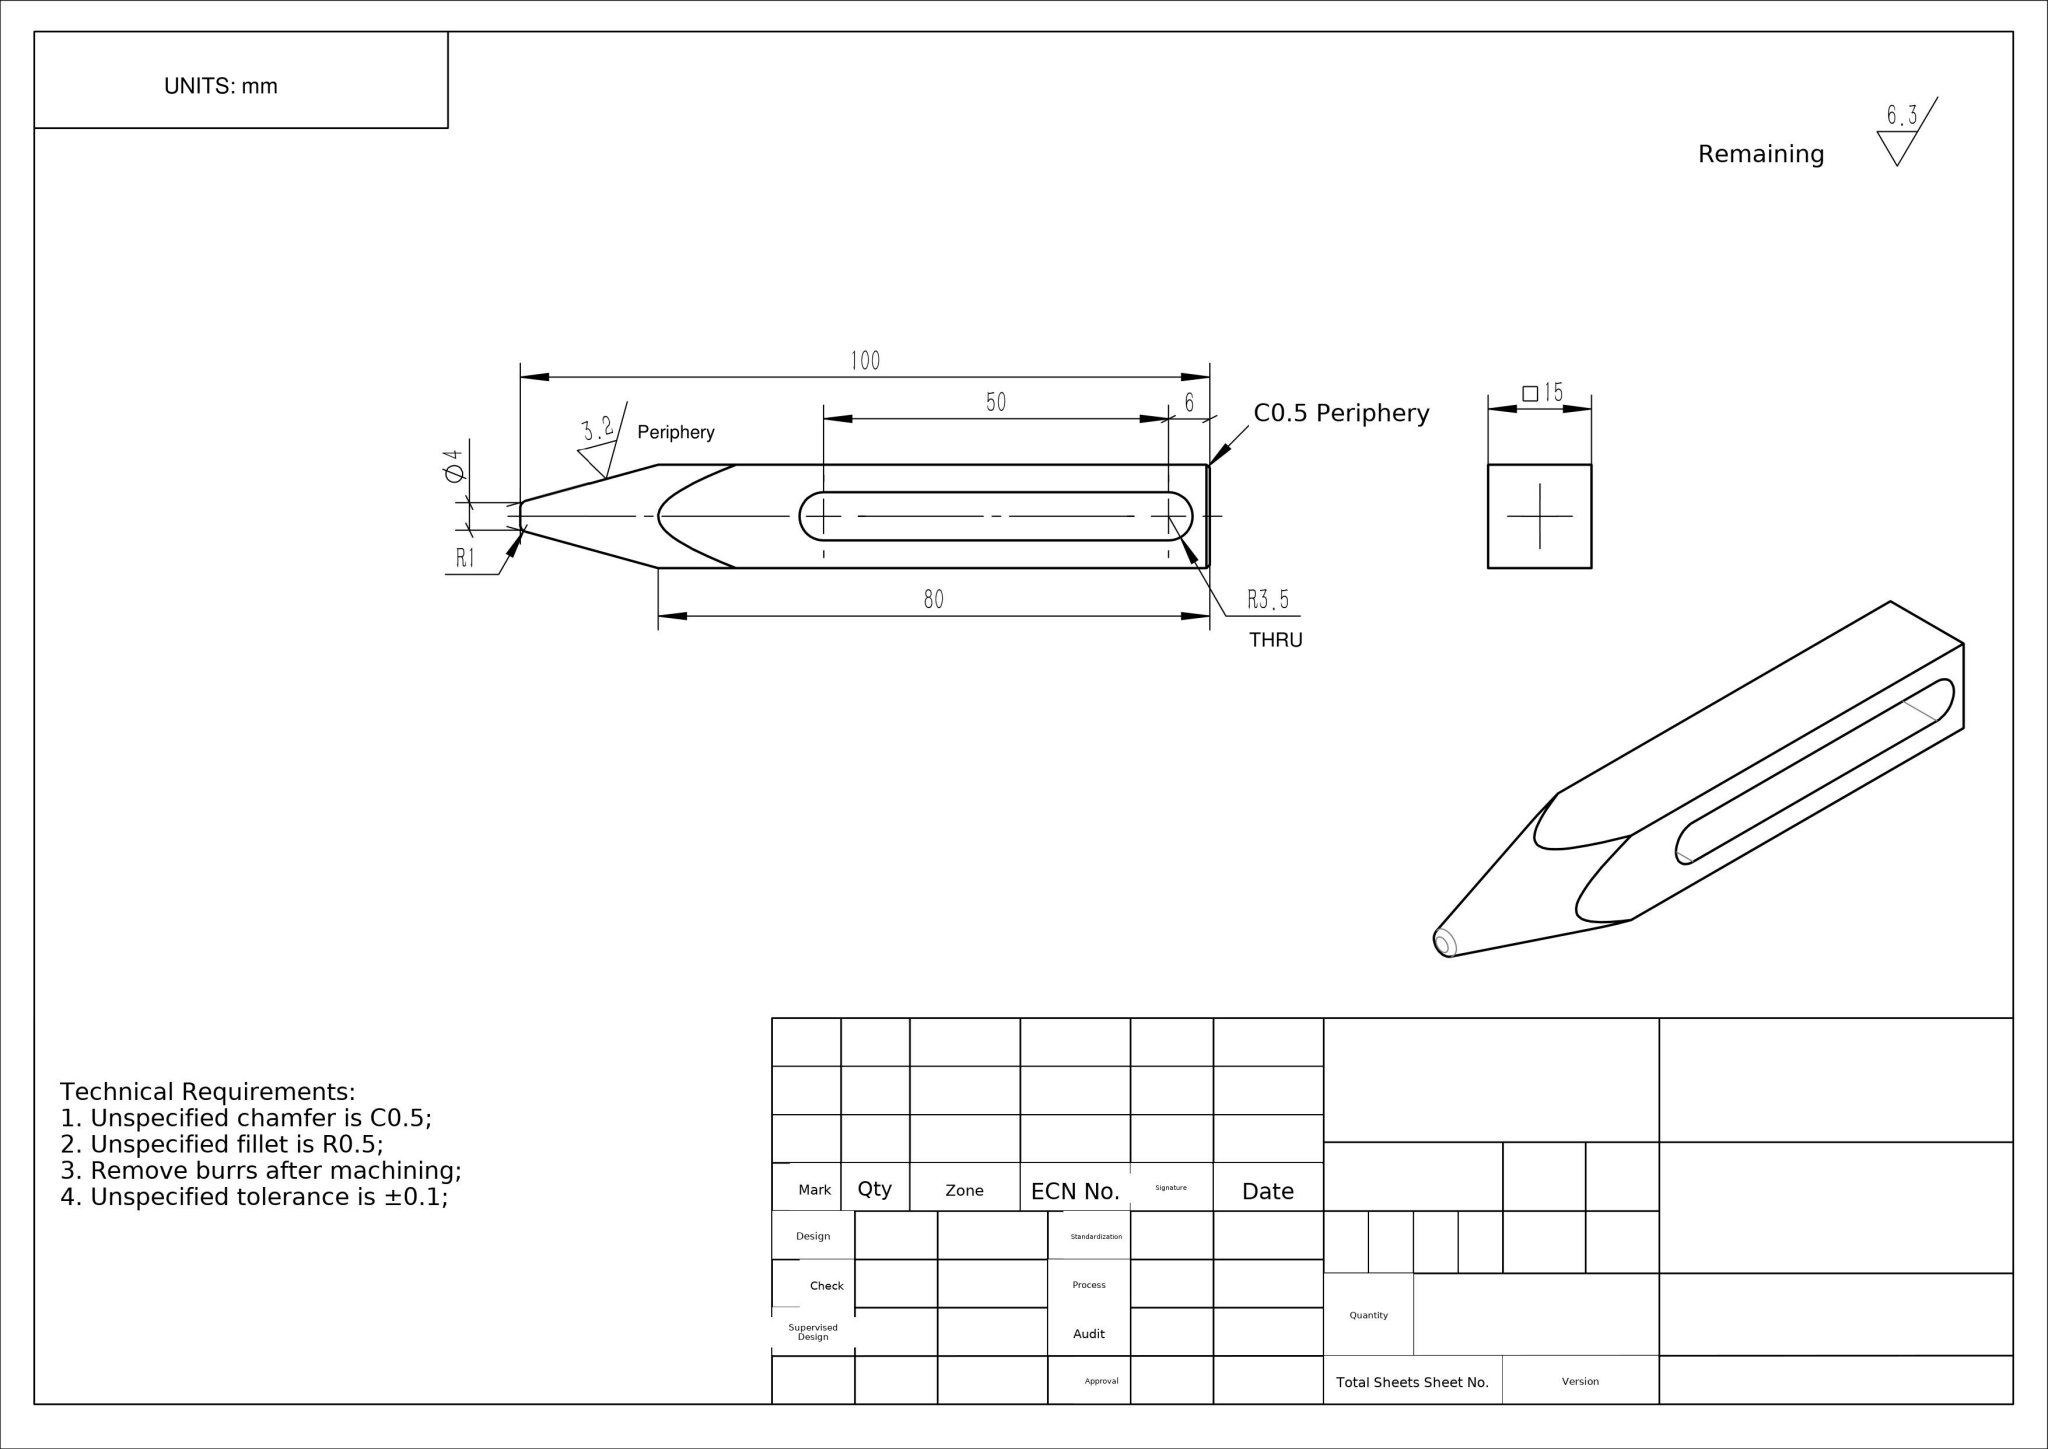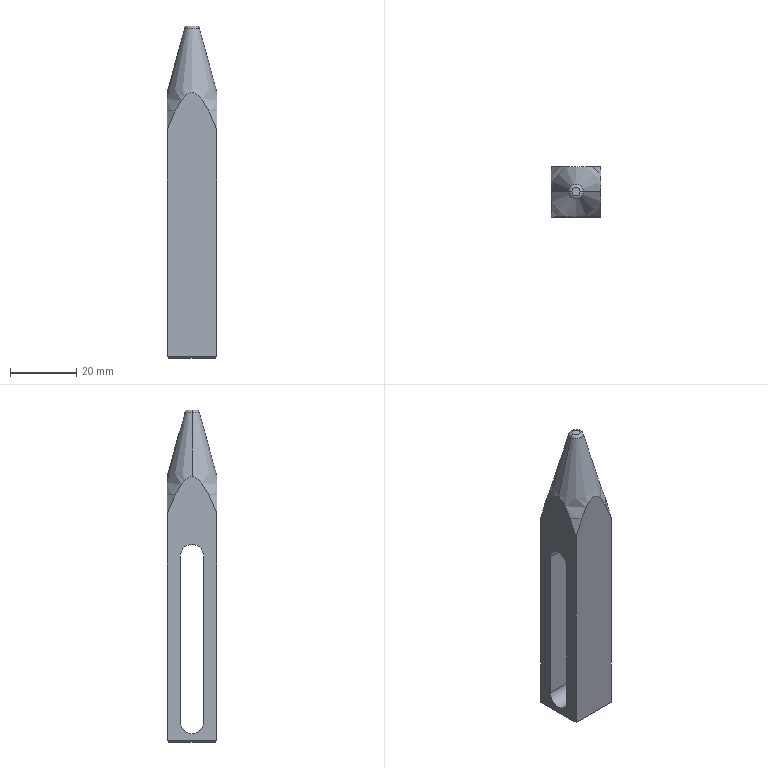Part | NX | mm | 1 solid | 19 faces | box 15 x 15 x 100 mm | volume 13574 mm3 | plane 12 | cylinder 3 | torus 2 | cone 2 | commonest cylinder face diameters 7 x3
STEP:
#1=COLOUR_RGB('',0.698,0.698,0.698);
#2=FILL_AREA_STYLE_COLOUR('',#1);
#3=FILL_AREA_STYLE('',(#2));
#4=SURFACE_STYLE_FILL_AREA(#3);
#5=SURFACE_SIDE_STYLE('',(#4));
#6=SURFACE_STYLE_USAGE(.BOTH.,#5);
#7=PRESENTATION_STYLE_ASSIGNMENT((#6));
#8=CARTESIAN_POINT('',(7.5,0.,9.5));
#9=VERTEX_POINT('',#8);
#10=CARTESIAN_POINT('',(7.5,3.5,6.));
#11=VERTEX_POINT('',#10);
#12=CARTESIAN_POINT('',(7.5,0.,6.));
#13=DIRECTION('',(-1.,0.,0.));
#14=DIRECTION('',(0.,0.,1.));
#15=AXIS2_PLACEMENT_3D('',#12,#13,#14);
#16=CIRCLE('',#15,3.5);
#17=EDGE_CURVE('',#9,#11,#16,.T.);
#18=ORIENTED_EDGE('',*,*,#17,.F.);
#19=CARTESIAN_POINT('',(-7.5,0.,9.5));
#20=VERTEX_POINT('',#19);
#21=CARTESIAN_POINT('',(7.5,0.,9.5));
#22=DIRECTION('',(-1.,0.,0.));
#23=VECTOR('',#22,1000.);
#24=LINE('',#21,#23);
#25=EDGE_CURVE('',#9,#20,#24,.T.);
#26=ORIENTED_EDGE('',*,*,#25,.T.);
#27=CARTESIAN_POINT('',(-7.5,3.5,6.));
#28=VERTEX_POINT('',#27);
#29=CARTESIAN_POINT('',(-7.5,0.,6.));
#30=DIRECTION('',(-1.,0.,0.));
#31=DIRECTION('',(0.,0.,1.));
#32=AXIS2_PLACEMENT_3D('',#29,#30,#31);
#33=CIRCLE('',#32,3.5);
#34=EDGE_CURVE('',#20,#28,#33,.T.);
#35=ORIENTED_EDGE('',*,*,#34,.T.);
#36=CARTESIAN_POINT('',(7.5,3.5,6.));
#37=DIRECTION('',(-1.,0.,0.));
#38=VECTOR('',#37,1000.);
#39=LINE('',#36,#38);
#40=EDGE_CURVE('',#11,#28,#39,.T.);
#41=ORIENTED_EDGE('',*,*,#40,.F.);
#42=EDGE_LOOP('',(#18,#26,#35,#41));
#43=FACE_OUTER_BOUND('',#42,.T.);
#44=CARTESIAN_POINT('',(7.5,0.,6.));
#45=DIRECTION('',(-1.,0.,0.));
#46=DIRECTION('',(0.,0.,1.));
#47=AXIS2_PLACEMENT_3D('',#44,#45,#46);
#48=CYLINDRICAL_SURFACE('',#47,3.5);
#49=ADVANCED_FACE('',(#43),#48,.F.);
#50=CARTESIAN_POINT('',(-2.202,0.,49.265));
#51=VERTEX_POINT('',#50);
#52=CARTESIAN_POINT('',(2.202,0.,49.265));
#53=VERTEX_POINT('',#52);
#54=CARTESIAN_POINT('',(0.,0.,49.265));
#55=DIRECTION('',(0.,0.,-1.));
#56=DIRECTION('',(-1.,0.,0.));
#57=AXIS2_PLACEMENT_3D('',#54,#55,#56);
#58=CIRCLE('',#57,2.202);
#59=EDGE_CURVE('',#51,#53,#58,.T.);
#60=ORIENTED_EDGE('',*,*,#59,.F.);
#61=CARTESIAN_POINT('',(-1.238,0.,50.));
#62=VERTEX_POINT('',#61);
#63=CARTESIAN_POINT('',(-1.238,0.,49.));
#64=DIRECTION('',(0.,1.,0.));
#65=DIRECTION('',(-1.,0.,0.));
#66=AXIS2_PLACEMENT_3D('',#63,#64,#65);
#67=CIRCLE('',#66,1.);
#68=EDGE_CURVE('',#51,#62,#67,.T.);
#69=ORIENTED_EDGE('',*,*,#68,.T.);
#70=CARTESIAN_POINT('',(1.238,0.,50.));
#71=VERTEX_POINT('',#70);
#72=CARTESIAN_POINT('',(0.,0.,50.));
#73=DIRECTION('',(0.,0.,1.));
#74=DIRECTION('',(1.,0.,0.));
#75=AXIS2_PLACEMENT_3D('',#72,#73,#74);
#76=CIRCLE('',#75,1.238);
#77=EDGE_CURVE('',#71,#62,#76,.T.);
#78=ORIENTED_EDGE('',*,*,#77,.F.);
#79=CARTESIAN_POINT('',(1.238,0.,49.));
#80=DIRECTION('',(0.,-1.,0.));
#81=DIRECTION('',(0.,0.,-1.));
#82=AXIS2_PLACEMENT_3D('',#79,#80,#81);
#83=CIRCLE('',#82,1.);
#84=EDGE_CURVE('',#53,#71,#83,.T.);
#85=ORIENTED_EDGE('',*,*,#84,.F.);
#86=EDGE_LOOP('',(#60,#69,#78,#85));
#87=FACE_OUTER_BOUND('',#86,.T.);
#88=CARTESIAN_POINT('',(0.,0.,49.));
#89=DIRECTION('',(0.,0.,1.));
#90=DIRECTION('',(1.,0.,0.));
#91=AXIS2_PLACEMENT_3D('',#88,#89,#90);
#92=TOROIDAL_SURFACE('',#91,1.238,1.);
#93=ADVANCED_FACE('',(#87),#92,.T.);
#94=ORIENTED_EDGE('',*,*,#59,.T.);
#95=CARTESIAN_POINT('',(7.5,0.,30.));
#96=VERTEX_POINT('',#95);
#97=CARTESIAN_POINT('',(12.,0.,13.636));
#98=DIRECTION('',(0.2652,0.,-0.9642));
#99=VECTOR('',#98,1000.);
#100=LINE('',#97,#99);
#101=EDGE_CURVE('',#53,#96,#100,.T.);
#102=ORIENTED_EDGE('',*,*,#101,.T.);
#103=CARTESIAN_POINT('',(7.5,7.5,18.703));
#104=VERTEX_POINT('',#103);
#105=CARTESIAN_POINT('',(7.5,7.5,18.703));
#106=CARTESIAN_POINT('',(7.5,7.077,19.79));
#107=CARTESIAN_POINT('',(7.5,6.64,20.871));
#108=CARTESIAN_POINT('',(7.5,5.714,23.011));
#109=CARTESIAN_POINT('',(7.5,5.228,24.07));
#110=CARTESIAN_POINT('',(7.5,4.421,25.626));
#111=CARTESIAN_POINT('',(7.5,4.139,26.139));
#112=CARTESIAN_POINT('',(7.5,3.53,27.146));
#113=CARTESIAN_POINT('',(7.5,3.207,27.637));
#114=CARTESIAN_POINT('',(7.5,2.669,28.33));
#115=CARTESIAN_POINT('',(7.5,2.482,28.555));
#116=CARTESIAN_POINT('',(7.5,2.078,28.981));
#117=CARTESIAN_POINT('',(7.5,1.861,29.186));
#118=CARTESIAN_POINT('',(7.5,1.392,29.546));
#119=CARTESIAN_POINT('',(7.5,1.142,29.704));
#120=CARTESIAN_POINT('',(7.5,0.7287,29.876));
#121=CARTESIAN_POINT('',(7.5,0.5877,29.921));
#122=CARTESIAN_POINT('',(7.5,0.2981,29.984));
#123=CARTESIAN_POINT('',(7.5,0.1479,30.));
#124=CARTESIAN_POINT('',(7.5,0.,30.));
#125=B_SPLINE_CURVE_WITH_KNOTS('',3,(#105,#106,#107,#108,#109,#110,#111,#112,#113,#114,#115,#116,#117,#118,#119,#120,#121,#122,#123,#124),.UNSPECIFIED.,.F.,.F.,(4,2,2,2,2,2,2,2,2,4),(0.05853,0.06203,0.06553,0.06728,0.06903,0.06991,0.07078,0.07166,0.0721,0.07253),.UNSPECIFIED.);
#126=EDGE_CURVE('',#104,#96,#125,.T.);
#127=ORIENTED_EDGE('',*,*,#126,.F.);
#128=CARTESIAN_POINT('',(-7.5,7.5,18.703));
#129=VERTEX_POINT('',#128);
#130=CARTESIAN_POINT('',(-7.5,7.5,18.703));
#131=CARTESIAN_POINT('',(-7.076,7.5,19.794));
#132=CARTESIAN_POINT('',(-6.636,7.5,20.881));
#133=CARTESIAN_POINT('',(-5.705,7.5,23.032));
#134=CARTESIAN_POINT('',(-5.215,7.5,24.098));
#135=CARTESIAN_POINT('',(-4.403,7.5,25.658));
#136=CARTESIAN_POINT('',(-4.121,7.5,26.17));
#137=CARTESIAN_POINT('',(-3.516,7.5,27.168));
#138=CARTESIAN_POINT('',(-3.194,7.5,27.655));
#139=CARTESIAN_POINT('',(-2.655,7.5,28.348));
#140=CARTESIAN_POINT('',(-2.466,7.5,28.573));
#141=CARTESIAN_POINT('',(-2.057,7.5,29.002));
#142=CARTESIAN_POINT('',(-1.841,7.5,29.203));
#143=CARTESIAN_POINT('',(-1.37,7.5,29.561));
#144=CARTESIAN_POINT('',(-1.117,7.5,29.716));
#145=CARTESIAN_POINT('',(-0.7103,7.5,29.882));
#146=CARTESIAN_POINT('',(-0.5681,7.5,29.927));
#147=CARTESIAN_POINT('',(-0.2766,7.5,29.987));
#148=CARTESIAN_POINT('',(-0.1298,7.5,30.001));
#149=CARTESIAN_POINT('',(0.1658,7.5,29.999));
#150=CARTESIAN_POINT('',(0.3156,7.5,29.981));
#151=CARTESIAN_POINT('',(0.6043,7.5,29.917));
#152=CARTESIAN_POINT('',(0.7448,7.5,29.87));
#153=CARTESIAN_POINT('',(1.156,7.5,29.696));
#154=CARTESIAN_POINT('',(1.406,7.5,29.537));
#155=CARTESIAN_POINT('',(1.872,7.5,29.175));
#156=CARTESIAN_POINT('',(2.089,7.5,28.971));
#157=CARTESIAN_POINT('',(2.491,7.5,28.544));
#158=CARTESIAN_POINT('',(2.678,7.5,28.32));
#159=CARTESIAN_POINT('',(3.214,7.5,27.626));
#160=CARTESIAN_POINT('',(3.537,7.5,27.136));
#161=CARTESIAN_POINT('',(4.144,7.5,26.13));
#162=CARTESIAN_POINT('',(4.425,7.5,25.618));
#163=CARTESIAN_POINT('',(5.231,7.5,24.063));
#164=CARTESIAN_POINT('',(5.717,7.5,23.005));
#165=CARTESIAN_POINT('',(6.641,7.5,20.868));
#166=CARTESIAN_POINT('',(7.078,7.5,19.789));
#167=CARTESIAN_POINT('',(7.5,7.5,18.703));
#168=B_SPLINE_CURVE_WITH_KNOTS('',3,(#130,#131,#132,#133,#134,#135,#136,#137,#138,#139,#140,#141,#142,#143,#144,#145,#146,#147,#148,#149,#150,#151,#152,#153,#154,#155,#156,#157,#158,#159,#160,#161,#162,#163,#164,#165,#166,#167),.UNSPECIFIED.,.F.,.F.,(4,2,2,2,2,2,2,2,2,2,2,2,2,2,2,2,2,2,4),(0.07672,0.08023,0.08374,0.0855,0.08725,0.08813,0.08901,0.08988,0.09032,0.09076,0.0912,0.09164,0.09252,0.09339,0.09427,0.09603,0.09778,0.1013,0.1048),.UNSPECIFIED.);
#169=EDGE_CURVE('',#129,#104,#168,.T.);
#170=ORIENTED_EDGE('',*,*,#169,.F.);
#171=CARTESIAN_POINT('',(-7.5,-0.,30.));
#172=VERTEX_POINT('',#171);
#173=CARTESIAN_POINT('',(-7.5,-0.,30.));
#174=CARTESIAN_POINT('',(-7.5,0.1479,30.));
#175=CARTESIAN_POINT('',(-7.5,0.2981,29.984));
#176=CARTESIAN_POINT('',(-7.5,0.5877,29.921));
#177=CARTESIAN_POINT('',(-7.5,0.7287,29.876));
#178=CARTESIAN_POINT('',(-7.5,1.142,29.704));
#179=CARTESIAN_POINT('',(-7.5,1.392,29.546));
#180=CARTESIAN_POINT('',(-7.5,1.861,29.186));
#181=CARTESIAN_POINT('',(-7.5,2.078,28.981));
#182=CARTESIAN_POINT('',(-7.5,2.482,28.555));
#183=CARTESIAN_POINT('',(-7.5,2.669,28.33));
#184=CARTESIAN_POINT('',(-7.5,3.207,27.637));
#185=CARTESIAN_POINT('',(-7.5,3.53,27.146));
#186=CARTESIAN_POINT('',(-7.5,4.139,26.139));
#187=CARTESIAN_POINT('',(-7.5,4.421,25.626));
#188=CARTESIAN_POINT('',(-7.5,5.228,24.07));
#189=CARTESIAN_POINT('',(-7.5,5.714,23.011));
#190=CARTESIAN_POINT('',(-7.5,6.64,20.871));
#191=CARTESIAN_POINT('',(-7.5,7.077,19.79));
#192=CARTESIAN_POINT('',(-7.5,7.5,18.703));
#193=B_SPLINE_CURVE_WITH_KNOTS('',3,(#173,#174,#175,#176,#177,#178,#179,#180,#181,#182,#183,#184,#185,#186,#187,#188,#189,#190,#191,#192),.UNSPECIFIED.,.F.,.F.,(4,2,2,2,2,2,2,2,2,4),(0.09074,0.09118,0.09162,0.0925,0.09338,0.09426,0.09602,0.09777,0.1013,0.1048),.UNSPECIFIED.);
#194=EDGE_CURVE('',#172,#129,#193,.T.);
#195=ORIENTED_EDGE('',*,*,#194,.F.);
#196=CARTESIAN_POINT('',(-12.,0.,13.636));
#197=DIRECTION('',(-0.2652,0.,-0.9642));
#198=VECTOR('',#197,1000.);
#199=LINE('',#196,#198);
#200=EDGE_CURVE('',#51,#172,#199,.T.);
#201=ORIENTED_EDGE('',*,*,#200,.F.);
#202=EDGE_LOOP('',(#94,#102,#127,#170,#195,#201));
#203=FACE_OUTER_BOUND('',#202,.T.);
#204=CARTESIAN_POINT('',(0.,0.,13.636));
#205=DIRECTION('',(0.,0.,-1.));
#206=DIRECTION('',(-1.,0.,0.));
#207=AXIS2_PLACEMENT_3D('',#204,#205,#206);
#208=CONICAL_SURFACE('',#207,12.,0.2684);
#209=ADVANCED_FACE('',(#203),#208,.T.);
#210=CARTESIAN_POINT('',(-7.5,-3.5,-44.));
#211=VERTEX_POINT('',#210);
#212=CARTESIAN_POINT('',(-7.5,-3.5,6.));
#213=VERTEX_POINT('',#212);
#214=CARTESIAN_POINT('',(-7.5,-3.5,-44.));
#215=DIRECTION('',(0.,0.,1.));
#216=VECTOR('',#215,1000.);
#217=LINE('',#214,#216);
#218=EDGE_CURVE('',#211,#213,#217,.T.);
#219=ORIENTED_EDGE('',*,*,#218,.F.);
#220=CARTESIAN_POINT('',(-7.5,3.5,-44.));
#221=VERTEX_POINT('',#220);
#222=CARTESIAN_POINT('',(-7.5,0.,-44.));
#223=DIRECTION('',(-1.,0.,0.));
#224=DIRECTION('',(0.,0.,1.));
#225=AXIS2_PLACEMENT_3D('',#222,#223,#224);
#226=CIRCLE('',#225,3.5);
#227=EDGE_CURVE('',#221,#211,#226,.T.);
#228=ORIENTED_EDGE('',*,*,#227,.F.);
#229=CARTESIAN_POINT('',(-7.5,3.5,-44.));
#230=DIRECTION('',(0.,0.,-1.));
#231=VECTOR('',#230,1000.);
#232=LINE('',#229,#231);
#233=EDGE_CURVE('',#28,#221,#232,.T.);
#234=ORIENTED_EDGE('',*,*,#233,.F.);
#235=ORIENTED_EDGE('',*,*,#34,.F.);
#236=CARTESIAN_POINT('',(-7.5,0.,6.));
#237=DIRECTION('',(-1.,0.,0.));
#238=DIRECTION('',(0.,0.,1.));
#239=AXIS2_PLACEMENT_3D('',#236,#237,#238);
#240=CIRCLE('',#239,3.5);
#241=EDGE_CURVE('',#213,#20,#240,.T.);
#242=ORIENTED_EDGE('',*,*,#241,.F.);
#243=EDGE_LOOP('',(#219,#228,#234,#235,#242));
#244=FACE_BOUND('',#243,.T.);
#245=CARTESIAN_POINT('',(-7.5,7.5,-49.5));
#246=VERTEX_POINT('',#245);
#247=CARTESIAN_POINT('',(-7.5,7.5,50.));
#248=DIRECTION('',(0.,0.,-1.));
#249=VECTOR('',#248,1000.);
#250=LINE('',#247,#249);
#251=EDGE_CURVE('',#129,#246,#250,.T.);
#252=ORIENTED_EDGE('',*,*,#251,.T.);
#253=CARTESIAN_POINT('',(-7.5,-7.5,-49.5));
#254=VERTEX_POINT('',#253);
#255=CARTESIAN_POINT('',(-7.5,-7.5,-49.5));
#256=DIRECTION('',(0.,-1.,0.));
#257=VECTOR('',#256,1000.);
#258=LINE('',#255,#257);
#259=EDGE_CURVE('',#246,#254,#258,.T.);
#260=ORIENTED_EDGE('',*,*,#259,.T.);
#261=CARTESIAN_POINT('',(-7.5,-7.5,18.703));
#262=VERTEX_POINT('',#261);
#263=CARTESIAN_POINT('',(-7.5,-7.5,50.));
#264=DIRECTION('',(0.,0.,-1.));
#265=VECTOR('',#264,1000.);
#266=LINE('',#263,#265);
#267=EDGE_CURVE('',#262,#254,#266,.T.);
#268=ORIENTED_EDGE('',*,*,#267,.F.);
#269=CARTESIAN_POINT('',(-7.5,-7.5,18.703));
#270=CARTESIAN_POINT('',(-7.5,-7.076,19.793));
#271=CARTESIAN_POINT('',(-7.5,-6.637,20.879));
#272=CARTESIAN_POINT('',(-7.5,-5.707,23.027));
#273=CARTESIAN_POINT('',(-7.5,-5.218,24.091));
#274=CARTESIAN_POINT('',(-7.5,-4.408,25.649));
#275=CARTESIAN_POINT('',(-7.5,-4.126,26.161));
#276=CARTESIAN_POINT('',(-7.5,-3.522,27.158));
#277=CARTESIAN_POINT('',(-7.5,-3.201,27.644));
#278=CARTESIAN_POINT('',(-7.5,-2.664,28.337));
#279=CARTESIAN_POINT('',(-7.5,-2.475,28.562));
#280=CARTESIAN_POINT('',(-7.5,-2.068,28.991));
#281=CARTESIAN_POINT('',(-7.5,-1.853,29.193));
#282=CARTESIAN_POINT('',(-7.5,-1.384,29.552));
#283=CARTESIAN_POINT('',(-7.5,-1.132,29.709));
#284=CARTESIAN_POINT('',(-7.5,-0.5912,29.933));
#285=CARTESIAN_POINT('',(-7.5,-0.295,30.));
#286=CARTESIAN_POINT('',(-7.5,-0.,30.));
#287=B_SPLINE_CURVE_WITH_KNOTS('',3,(#269,#270,#271,#272,#273,#274,#275,#276,#277,#278,#279,#280,#281,#282,#283,#284,#285,#286),.UNSPECIFIED.,.F.,.F.,(4,2,2,2,2,2,2,2,4),(0.07672,0.08023,0.08373,0.08549,0.08724,0.08812,0.08899,0.08987,0.09074),.UNSPECIFIED.);
#288=EDGE_CURVE('',#262,#172,#287,.T.);
#289=ORIENTED_EDGE('',*,*,#288,.T.);
#290=ORIENTED_EDGE('',*,*,#194,.T.);
#291=EDGE_LOOP('',(#252,#260,#268,#289,#290));
#292=FACE_OUTER_BOUND('',#291,.T.);
#293=CARTESIAN_POINT('',(-7.5,-7.5,50.));
#294=DIRECTION('',(1.,0.,0.));
#295=DIRECTION('',(0.,0.,-1.));
#296=AXIS2_PLACEMENT_3D('',#293,#294,#295);
#297=PLANE('',#296);
#298=ADVANCED_FACE('',(#244,#292),#297,.F.);
#299=ORIENTED_EDGE('',*,*,#267,.T.);
#300=CARTESIAN_POINT('',(7.5,-7.5,-49.5));
#301=VERTEX_POINT('',#300);
#302=CARTESIAN_POINT('',(7.5,-7.5,-49.5));
#303=DIRECTION('',(1.,0.,0.));
#304=VECTOR('',#303,1000.);
#305=LINE('',#302,#304);
#306=EDGE_CURVE('',#254,#301,#305,.T.);
#307=ORIENTED_EDGE('',*,*,#306,.T.);
#308=CARTESIAN_POINT('',(7.5,-7.5,18.703));
#309=VERTEX_POINT('',#308);
#310=CARTESIAN_POINT('',(7.5,-7.5,50.));
#311=DIRECTION('',(0.,0.,-1.));
#312=VECTOR('',#311,1000.);
#313=LINE('',#310,#312);
#314=EDGE_CURVE('',#309,#301,#313,.T.);
#315=ORIENTED_EDGE('',*,*,#314,.F.);
#316=CARTESIAN_POINT('',(7.5,-7.5,18.703));
#317=CARTESIAN_POINT('',(7.078,-7.5,19.789));
#318=CARTESIAN_POINT('',(6.641,-7.5,20.868));
#319=CARTESIAN_POINT('',(5.717,-7.5,23.005));
#320=CARTESIAN_POINT('',(5.231,-7.5,24.063));
#321=CARTESIAN_POINT('',(4.425,-7.5,25.618));
#322=CARTESIAN_POINT('',(4.144,-7.5,26.13));
#323=CARTESIAN_POINT('',(3.537,-7.5,27.136));
#324=CARTESIAN_POINT('',(3.214,-7.5,27.626));
#325=CARTESIAN_POINT('',(2.678,-7.5,28.32));
#326=CARTESIAN_POINT('',(2.491,-7.5,28.544));
#327=CARTESIAN_POINT('',(2.089,-7.5,28.971));
#328=CARTESIAN_POINT('',(1.872,-7.5,29.175));
#329=CARTESIAN_POINT('',(1.406,-7.5,29.537));
#330=CARTESIAN_POINT('',(1.156,-7.5,29.696));
#331=CARTESIAN_POINT('',(0.7448,-7.5,29.87));
#332=CARTESIAN_POINT('',(0.6043,-7.5,29.917));
#333=CARTESIAN_POINT('',(0.3156,-7.5,29.981));
#334=CARTESIAN_POINT('',(0.1658,-7.5,29.999));
#335=CARTESIAN_POINT('',(-0.1298,-7.5,30.001));
#336=CARTESIAN_POINT('',(-0.2766,-7.5,29.987));
#337=CARTESIAN_POINT('',(-0.5681,-7.5,29.927));
#338=CARTESIAN_POINT('',(-0.7103,-7.5,29.882));
#339=CARTESIAN_POINT('',(-1.117,-7.5,29.716));
#340=CARTESIAN_POINT('',(-1.37,-7.5,29.561));
#341=CARTESIAN_POINT('',(-1.841,-7.5,29.203));
#342=CARTESIAN_POINT('',(-2.057,-7.5,29.002));
#343=CARTESIAN_POINT('',(-2.466,-7.5,28.573));
#344=CARTESIAN_POINT('',(-2.655,-7.5,28.348));
#345=CARTESIAN_POINT('',(-3.194,-7.5,27.655));
#346=CARTESIAN_POINT('',(-3.516,-7.5,27.168));
#347=CARTESIAN_POINT('',(-4.121,-7.5,26.17));
#348=CARTESIAN_POINT('',(-4.403,-7.5,25.658));
#349=CARTESIAN_POINT('',(-5.215,-7.5,24.098));
#350=CARTESIAN_POINT('',(-5.705,-7.5,23.032));
#351=CARTESIAN_POINT('',(-6.636,-7.5,20.881));
#352=CARTESIAN_POINT('',(-7.076,-7.5,19.794));
#353=CARTESIAN_POINT('',(-7.5,-7.5,18.703));
#354=B_SPLINE_CURVE_WITH_KNOTS('',3,(#316,#317,#318,#319,#320,#321,#322,#323,#324,#325,#326,#327,#328,#329,#330,#331,#332,#333,#334,#335,#336,#337,#338,#339,#340,#341,#342,#343,#344,#345,#346,#347,#348,#349,#350,#351,#352,#353),.UNSPECIFIED.,.F.,.F.,(4,2,2,2,2,2,2,2,2,2,2,2,2,2,2,2,2,2,4),(0.05853,0.06203,0.06552,0.06727,0.06902,0.06989,0.07077,0.07164,0.07208,0.07252,0.07295,0.07339,0.07426,0.07514,0.07601,0.07776,0.07951,0.083,0.0865),.UNSPECIFIED.);
#355=EDGE_CURVE('',#309,#262,#354,.T.);
#356=ORIENTED_EDGE('',*,*,#355,.T.);
#357=EDGE_LOOP('',(#299,#307,#315,#356));
#358=FACE_OUTER_BOUND('',#357,.T.);
#359=CARTESIAN_POINT('',(7.5,-7.5,50.));
#360=DIRECTION('',(-0.,1.,0.));
#361=DIRECTION('',(-1.,-0.,0.));
#362=AXIS2_PLACEMENT_3D('',#359,#360,#361);
#363=PLANE('',#362);
#364=ADVANCED_FACE('',(#358),#363,.F.);
#365=CARTESIAN_POINT('',(7.5,3.5,-44.));
#366=VERTEX_POINT('',#365);
#367=CARTESIAN_POINT('',(7.5,3.5,-44.));
#368=DIRECTION('',(0.,0.,-1.));
#369=VECTOR('',#368,1000.);
#370=LINE('',#367,#369);
#371=EDGE_CURVE('',#11,#366,#370,.T.);
#372=ORIENTED_EDGE('',*,*,#371,.T.);
#373=CARTESIAN_POINT('',(7.5,-3.5,-44.));
#374=VERTEX_POINT('',#373);
#375=CARTESIAN_POINT('',(7.5,0.,-44.));
#376=DIRECTION('',(-1.,0.,0.));
#377=DIRECTION('',(0.,0.,1.));
#378=AXIS2_PLACEMENT_3D('',#375,#376,#377);
#379=CIRCLE('',#378,3.5);
#380=EDGE_CURVE('',#366,#374,#379,.T.);
#381=ORIENTED_EDGE('',*,*,#380,.T.);
#382=CARTESIAN_POINT('',(7.5,-3.5,6.));
#383=VERTEX_POINT('',#382);
#384=CARTESIAN_POINT('',(7.5,-3.5,-44.));
#385=DIRECTION('',(0.,0.,1.));
#386=VECTOR('',#385,1000.);
#387=LINE('',#384,#386);
#388=EDGE_CURVE('',#374,#383,#387,.T.);
#389=ORIENTED_EDGE('',*,*,#388,.T.);
#390=CARTESIAN_POINT('',(7.5,0.,6.));
#391=DIRECTION('',(-1.,0.,0.));
#392=DIRECTION('',(0.,0.,1.));
#393=AXIS2_PLACEMENT_3D('',#390,#391,#392);
#394=CIRCLE('',#393,3.5);
#395=EDGE_CURVE('',#383,#9,#394,.T.);
#396=ORIENTED_EDGE('',*,*,#395,.T.);
#397=ORIENTED_EDGE('',*,*,#17,.T.);
#398=EDGE_LOOP('',(#372,#381,#389,#396,#397));
#399=FACE_BOUND('',#398,.T.);
#400=ORIENTED_EDGE('',*,*,#314,.T.);
#401=CARTESIAN_POINT('',(7.5,7.5,-49.5));
#402=VERTEX_POINT('',#401);
#403=CARTESIAN_POINT('',(7.5,-7.5,-49.5));
#404=DIRECTION('',(0.,1.,0.));
#405=VECTOR('',#404,1000.);
#406=LINE('',#403,#405);
#407=EDGE_CURVE('',#301,#402,#406,.T.);
#408=ORIENTED_EDGE('',*,*,#407,.T.);
#409=CARTESIAN_POINT('',(7.5,7.5,50.));
#410=DIRECTION('',(0.,0.,-1.));
#411=VECTOR('',#410,1000.);
#412=LINE('',#409,#411);
#413=EDGE_CURVE('',#104,#402,#412,.T.);
#414=ORIENTED_EDGE('',*,*,#413,.F.);
#415=ORIENTED_EDGE('',*,*,#126,.T.);
#416=CARTESIAN_POINT('',(7.5,0.,30.));
#417=CARTESIAN_POINT('',(7.5,-0.295,30.));
#418=CARTESIAN_POINT('',(7.5,-0.5912,29.933));
#419=CARTESIAN_POINT('',(7.5,-1.132,29.709));
#420=CARTESIAN_POINT('',(7.5,-1.384,29.552));
#421=CARTESIAN_POINT('',(7.5,-1.853,29.193));
#422=CARTESIAN_POINT('',(7.5,-2.068,28.991));
#423=CARTESIAN_POINT('',(7.5,-2.475,28.562));
#424=CARTESIAN_POINT('',(7.5,-2.664,28.337));
#425=CARTESIAN_POINT('',(7.5,-3.201,27.644));
#426=CARTESIAN_POINT('',(7.5,-3.522,27.158));
#427=CARTESIAN_POINT('',(7.5,-4.126,26.161));
#428=CARTESIAN_POINT('',(7.5,-4.408,25.649));
#429=CARTESIAN_POINT('',(7.5,-5.218,24.091));
#430=CARTESIAN_POINT('',(7.5,-5.707,23.027));
#431=CARTESIAN_POINT('',(7.5,-6.637,20.879));
#432=CARTESIAN_POINT('',(7.5,-7.076,19.793));
#433=CARTESIAN_POINT('',(7.5,-7.5,18.703));
#434=B_SPLINE_CURVE_WITH_KNOTS('',3,(#416,#417,#418,#419,#420,#421,#422,#423,#424,#425,#426,#427,#428,#429,#430,#431,#432,#433),.UNSPECIFIED.,.F.,.F.,(4,2,2,2,2,2,2,2,4),(0.07253,0.07341,0.07428,0.07515,0.07603,0.07777,0.07952,0.08301,0.0865),.UNSPECIFIED.);
#435=EDGE_CURVE('',#96,#309,#434,.T.);
#436=ORIENTED_EDGE('',*,*,#435,.T.);
#437=EDGE_LOOP('',(#400,#408,#414,#415,#436));
#438=FACE_OUTER_BOUND('',#437,.T.);
#439=CARTESIAN_POINT('',(7.5,-7.5,50.));
#440=DIRECTION('',(-1.,0.,0.));
#441=DIRECTION('',(0.,0.,1.));
#442=AXIS2_PLACEMENT_3D('',#439,#440,#441);
#443=PLANE('',#442);
#444=ADVANCED_FACE('',(#399,#438),#443,.F.);
#445=ORIENTED_EDGE('',*,*,#413,.T.);
#446=CARTESIAN_POINT('',(7.5,7.5,-49.5));
#447=DIRECTION('',(-1.,-0.,0.));
#448=VECTOR('',#447,1000.);
#449=LINE('',#446,#448);
#450=EDGE_CURVE('',#402,#246,#449,.T.);
#451=ORIENTED_EDGE('',*,*,#450,.T.);
#452=ORIENTED_EDGE('',*,*,#251,.F.);
#453=ORIENTED_EDGE('',*,*,#169,.T.);
#454=EDGE_LOOP('',(#445,#451,#452,#453));
#455=FACE_OUTER_BOUND('',#454,.T.);
#456=CARTESIAN_POINT('',(7.5,7.5,50.));
#457=DIRECTION('',(0.,-1.,0.));
#458=DIRECTION('',(1.,0.,0.));
#459=AXIS2_PLACEMENT_3D('',#456,#457,#458);
#460=PLANE('',#459);
#461=ADVANCED_FACE('',(#455),#460,.F.);
#462=CARTESIAN_POINT('',(7.,7.,-50.));
#463=VERTEX_POINT('',#462);
#464=CARTESIAN_POINT('',(7.,-7.,-50.));
#465=VERTEX_POINT('',#464);
#466=CARTESIAN_POINT('',(7.,0.,-50.));
#467=DIRECTION('',(0.,-1.,0.));
#468=VECTOR('',#467,1000.);
#469=LINE('',#466,#468);
#470=EDGE_CURVE('',#463,#465,#469,.T.);
#471=ORIENTED_EDGE('',*,*,#470,.T.);
#472=CARTESIAN_POINT('',(-7.,-7.,-50.));
#473=VERTEX_POINT('',#472);
#474=CARTESIAN_POINT('',(0.,-7.,-50.));
#475=DIRECTION('',(-1.,-0.,0.));
#476=VECTOR('',#475,1000.);
#477=LINE('',#474,#476);
#478=EDGE_CURVE('',#465,#473,#477,.T.);
#479=ORIENTED_EDGE('',*,*,#478,.T.);
#480=CARTESIAN_POINT('',(-7.,7.,-50.));
#481=VERTEX_POINT('',#480);
#482=CARTESIAN_POINT('',(-7.,0.,-50.));
#483=DIRECTION('',(0.,1.,0.));
#484=VECTOR('',#483,1000.);
#485=LINE('',#482,#484);
#486=EDGE_CURVE('',#473,#481,#485,.T.);
#487=ORIENTED_EDGE('',*,*,#486,.T.);
#488=CARTESIAN_POINT('',(-0.,7.,-50.));
#489=DIRECTION('',(1.,0.,0.));
#490=VECTOR('',#489,1000.);
#491=LINE('',#488,#490);
#492=EDGE_CURVE('',#481,#463,#491,.T.);
#493=ORIENTED_EDGE('',*,*,#492,.T.);
#494=EDGE_LOOP('',(#471,#479,#487,#493));
#495=FACE_OUTER_BOUND('',#494,.T.);
#496=CARTESIAN_POINT('',(0.,0.,-50.));
#497=DIRECTION('',(0.,0.,1.));
#498=DIRECTION('',(1.,0.,0.));
#499=AXIS2_PLACEMENT_3D('',#496,#497,#498);
#500=PLANE('',#499);
#501=ADVANCED_FACE('',(#495),#500,.F.);
#502=ORIENTED_EDGE('',*,*,#101,.F.);
#503=CARTESIAN_POINT('',(0.,0.,49.265));
#504=DIRECTION('',(0.,0.,-1.));
#505=DIRECTION('',(-1.,0.,0.));
#506=AXIS2_PLACEMENT_3D('',#503,#504,#505);
#507=CIRCLE('',#506,2.202);
#508=EDGE_CURVE('',#53,#51,#507,.T.);
#509=ORIENTED_EDGE('',*,*,#508,.T.);
#510=ORIENTED_EDGE('',*,*,#200,.T.);
#511=ORIENTED_EDGE('',*,*,#288,.F.);
#512=ORIENTED_EDGE('',*,*,#355,.F.);
#513=ORIENTED_EDGE('',*,*,#435,.F.);
#514=EDGE_LOOP('',(#502,#509,#510,#511,#512,#513));
#515=FACE_OUTER_BOUND('',#514,.T.);
#516=CARTESIAN_POINT('',(0.,0.,13.636));
#517=DIRECTION('',(0.,0.,-1.));
#518=DIRECTION('',(-1.,0.,0.));
#519=AXIS2_PLACEMENT_3D('',#516,#517,#518);
#520=CONICAL_SURFACE('',#519,12.,0.2684);
#521=ADVANCED_FACE('',(#515),#520,.T.);
#522=ORIENTED_EDGE('',*,*,#77,.T.);
#523=CARTESIAN_POINT('',(0.,0.,50.));
#524=DIRECTION('',(0.,0.,1.));
#525=DIRECTION('',(1.,0.,0.));
#526=AXIS2_PLACEMENT_3D('',#523,#524,#525);
#527=CIRCLE('',#526,1.238);
#528=EDGE_CURVE('',#62,#71,#527,.T.);
#529=ORIENTED_EDGE('',*,*,#528,.T.);
#530=EDGE_LOOP('',(#522,#529));
#531=FACE_OUTER_BOUND('',#530,.T.);
#532=CARTESIAN_POINT('',(0.,0.,50.));
#533=DIRECTION('',(0.,0.,1.));
#534=DIRECTION('',(1.,0.,0.));
#535=AXIS2_PLACEMENT_3D('',#532,#533,#534);
#536=PLANE('',#535);
#537=ADVANCED_FACE('',(#531),#536,.T.);
#538=ORIENTED_EDGE('',*,*,#68,.F.);
#539=ORIENTED_EDGE('',*,*,#508,.F.);
#540=ORIENTED_EDGE('',*,*,#84,.T.);
#541=ORIENTED_EDGE('',*,*,#528,.F.);
#542=EDGE_LOOP('',(#538,#539,#540,#541));
#543=FACE_OUTER_BOUND('',#542,.T.);
#544=CARTESIAN_POINT('',(0.,0.,49.));
#545=DIRECTION('',(0.,0.,1.));
#546=DIRECTION('',(1.,0.,0.));
#547=AXIS2_PLACEMENT_3D('',#544,#545,#546);
#548=TOROIDAL_SURFACE('',#547,1.238,1.);
#549=ADVANCED_FACE('',(#543),#548,.T.);
#550=CARTESIAN_POINT('',(7.5,7.5,-49.5));
#551=DIRECTION('',(0.5774,0.5774,0.5774));
#552=VECTOR('',#551,1000.);
#553=LINE('',#550,#552);
#554=EDGE_CURVE('',#463,#402,#553,.T.);
#555=ORIENTED_EDGE('',*,*,#554,.F.);
#556=ORIENTED_EDGE('',*,*,#492,.F.);
#557=CARTESIAN_POINT('',(-2.5,2.5,-54.5));
#558=DIRECTION('',(0.5774,-0.5774,-0.5774));
#559=VECTOR('',#558,1000.);
#560=LINE('',#557,#559);
#561=EDGE_CURVE('',#246,#481,#560,.T.);
#562=ORIENTED_EDGE('',*,*,#561,.F.);
#563=ORIENTED_EDGE('',*,*,#450,.F.);
#564=EDGE_LOOP('',(#555,#556,#562,#563));
#565=FACE_OUTER_BOUND('',#564,.T.);
#566=CARTESIAN_POINT('',(7.5,7.5,-49.5));
#567=DIRECTION('',(0.,-0.7071,0.7071));
#568=DIRECTION('',(-1.,-0.,0.));
#569=AXIS2_PLACEMENT_3D('',#566,#567,#568);
#570=PLANE('',#569);
#571=ADVANCED_FACE('',(#565),#570,.F.);
#572=ORIENTED_EDGE('',*,*,#561,.T.);
#573=ORIENTED_EDGE('',*,*,#486,.F.);
#574=CARTESIAN_POINT('',(-7.5,-7.5,-49.5));
#575=DIRECTION('',(0.5774,0.5774,-0.5774));
#576=VECTOR('',#575,1000.);
#577=LINE('',#574,#576);
#578=EDGE_CURVE('',#254,#473,#577,.T.);
#579=ORIENTED_EDGE('',*,*,#578,.F.);
#580=ORIENTED_EDGE('',*,*,#259,.F.);
#581=EDGE_LOOP('',(#572,#573,#579,#580));
#582=FACE_OUTER_BOUND('',#581,.T.);
#583=CARTESIAN_POINT('',(-7.5,-7.5,-49.5));
#584=DIRECTION('',(0.7071,0.,0.7071));
#585=DIRECTION('',(0.,-1.,0.));
#586=AXIS2_PLACEMENT_3D('',#583,#584,#585);
#587=PLANE('',#586);
#588=ADVANCED_FACE('',(#582),#587,.F.);
#589=ORIENTED_EDGE('',*,*,#554,.T.);
#590=ORIENTED_EDGE('',*,*,#407,.F.);
#591=CARTESIAN_POINT('',(7.5,-7.5,-49.5));
#592=DIRECTION('',(0.5774,-0.5774,0.5774));
#593=VECTOR('',#592,1000.);
#594=LINE('',#591,#593);
#595=EDGE_CURVE('',#465,#301,#594,.T.);
#596=ORIENTED_EDGE('',*,*,#595,.F.);
#597=ORIENTED_EDGE('',*,*,#470,.F.);
#598=EDGE_LOOP('',(#589,#590,#596,#597));
#599=FACE_OUTER_BOUND('',#598,.T.);
#600=CARTESIAN_POINT('',(7.5,-7.5,-49.5));
#601=DIRECTION('',(-0.7071,0.,0.7071));
#602=DIRECTION('',(0.,1.,0.));
#603=AXIS2_PLACEMENT_3D('',#600,#601,#602);
#604=PLANE('',#603);
#605=ADVANCED_FACE('',(#599),#604,.F.);
#606=ORIENTED_EDGE('',*,*,#578,.T.);
#607=ORIENTED_EDGE('',*,*,#478,.F.);
#608=ORIENTED_EDGE('',*,*,#595,.T.);
#609=ORIENTED_EDGE('',*,*,#306,.F.);
#610=EDGE_LOOP('',(#606,#607,#608,#609));
#611=FACE_OUTER_BOUND('',#610,.T.);
#612=CARTESIAN_POINT('',(7.5,-7.5,-49.5));
#613=DIRECTION('',(-0.,0.7071,0.7071));
#614=DIRECTION('',(1.,0.,0.));
#615=AXIS2_PLACEMENT_3D('',#612,#613,#614);
#616=PLANE('',#615);
#617=ADVANCED_FACE('',(#611),#616,.F.);
#618=ORIENTED_EDGE('',*,*,#227,.T.);
#619=CARTESIAN_POINT('',(7.5,-3.5,-44.));
#620=DIRECTION('',(-1.,0.,0.));
#621=VECTOR('',#620,1000.);
#622=LINE('',#619,#621);
#623=EDGE_CURVE('',#374,#211,#622,.T.);
#624=ORIENTED_EDGE('',*,*,#623,.F.);
#625=ORIENTED_EDGE('',*,*,#380,.F.);
#626=CARTESIAN_POINT('',(7.5,3.5,-44.));
#627=DIRECTION('',(-1.,0.,0.));
#628=VECTOR('',#627,1000.);
#629=LINE('',#626,#628);
#630=EDGE_CURVE('',#366,#221,#629,.T.);
#631=ORIENTED_EDGE('',*,*,#630,.T.);
#632=EDGE_LOOP('',(#618,#624,#625,#631));
#633=FACE_OUTER_BOUND('',#632,.T.);
#634=CARTESIAN_POINT('',(7.5,0.,-44.));
#635=DIRECTION('',(-1.,0.,0.));
#636=DIRECTION('',(0.,0.,1.));
#637=AXIS2_PLACEMENT_3D('',#634,#635,#636);
#638=CYLINDRICAL_SURFACE('',#637,3.5);
#639=ADVANCED_FACE('',(#633),#638,.F.);
#640=ORIENTED_EDGE('',*,*,#233,.T.);
#641=ORIENTED_EDGE('',*,*,#630,.F.);
#642=ORIENTED_EDGE('',*,*,#371,.F.);
#643=ORIENTED_EDGE('',*,*,#40,.T.);
#644=EDGE_LOOP('',(#640,#641,#642,#643));
#645=FACE_OUTER_BOUND('',#644,.T.);
#646=CARTESIAN_POINT('',(7.5,3.5,-44.));
#647=DIRECTION('',(0.,1.,0.));
#648=DIRECTION('',(0.,0.,1.));
#649=AXIS2_PLACEMENT_3D('',#646,#647,#648);
#650=PLANE('',#649);
#651=ADVANCED_FACE('',(#645),#650,.F.);
#652=ORIENTED_EDGE('',*,*,#25,.F.);
#653=ORIENTED_EDGE('',*,*,#395,.F.);
#654=CARTESIAN_POINT('',(7.5,-3.5,6.));
#655=DIRECTION('',(-1.,0.,0.));
#656=VECTOR('',#655,1000.);
#657=LINE('',#654,#656);
#658=EDGE_CURVE('',#383,#213,#657,.T.);
#659=ORIENTED_EDGE('',*,*,#658,.T.);
#660=ORIENTED_EDGE('',*,*,#241,.T.);
#661=EDGE_LOOP('',(#652,#653,#659,#660));
#662=FACE_OUTER_BOUND('',#661,.T.);
#663=CARTESIAN_POINT('',(7.5,0.,6.));
#664=DIRECTION('',(-1.,0.,0.));
#665=DIRECTION('',(0.,0.,1.));
#666=AXIS2_PLACEMENT_3D('',#663,#664,#665);
#667=CYLINDRICAL_SURFACE('',#666,3.5);
#668=ADVANCED_FACE('',(#662),#667,.F.);
#669=ORIENTED_EDGE('',*,*,#218,.T.);
#670=ORIENTED_EDGE('',*,*,#658,.F.);
#671=ORIENTED_EDGE('',*,*,#388,.F.);
#672=ORIENTED_EDGE('',*,*,#623,.T.);
#673=EDGE_LOOP('',(#669,#670,#671,#672));
#674=FACE_OUTER_BOUND('',#673,.T.);
#675=CARTESIAN_POINT('',(7.5,-3.5,-44.));
#676=DIRECTION('',(0.,-1.,0.));
#677=DIRECTION('',(0.,0.,-1.));
#678=AXIS2_PLACEMENT_3D('',#675,#676,#677);
#679=PLANE('',#678);
#680=ADVANCED_FACE('',(#674),#679,.F.);
#681=CLOSED_SHELL('',(#49,#93,#209,#298,#364,#444,#461,#501,#521,#537,#549,#571,#588,#605,#617,#639,#651,#668,#680));
#682=MANIFOLD_SOLID_BREP('',#681);
#683=STYLED_ITEM('',(#7),#682);
#684=(LENGTH_UNIT()NAMED_UNIT(*)SI_UNIT(.MILLI.,.METRE.));
#685=UNCERTAINTY_MEASURE_WITH_UNIT(LENGTH_MEASURE(0.00001),#684,'','');
#686=(NAMED_UNIT(*)PLANE_ANGLE_UNIT()SI_UNIT($,.RADIAN.));
#687=(NAMED_UNIT(*)SI_UNIT($,.STERADIAN.)SOLID_ANGLE_UNIT());
#688=(GEOMETRIC_REPRESENTATION_CONTEXT(3)GLOBAL_UNCERTAINTY_ASSIGNED_CONTEXT((#685))GLOBAL_UNIT_ASSIGNED_CONTEXT((#684,#686,#687))REPRESENTATION_CONTEXT('',''));
#689=MECHANICAL_DESIGN_GEOMETRIC_PRESENTATION_REPRESENTATION('',(#683),#688);
#690=PRESENTATION_LAYER_ASSIGNMENT('','',(#683));
#691=COLOUR_RGB('',0.698,0.698,0.698);
#692=FILL_AREA_STYLE_COLOUR('',#691);
#693=FILL_AREA_STYLE('',(#692));
#694=SURFACE_STYLE_FILL_AREA(#693);
#695=SURFACE_SIDE_STYLE('',(#694));
#696=SURFACE_STYLE_USAGE(.BOTH.,#695);
#697=PRESENTATION_STYLE_ASSIGNMENT((#696));
#698=CARTESIAN_POINT('',(0.,0.,0.));
#699=DIRECTION('',(0.,0.,1.));
#700=DIRECTION('',(1.,0.,0.));
#701=AXIS2_PLACEMENT_3D('',#698,#699,#700);
#702=(LENGTH_UNIT()NAMED_UNIT(*)SI_UNIT(.MILLI.,.METRE.));
#703=UNCERTAINTY_MEASURE_WITH_UNIT(LENGTH_MEASURE(0.00001),#702,'','');
#704=(NAMED_UNIT(*)PLANE_ANGLE_UNIT()SI_UNIT($,.RADIAN.));
#705=(NAMED_UNIT(*)SI_UNIT($,.STERADIAN.)SOLID_ANGLE_UNIT());
#706=(GEOMETRIC_REPRESENTATION_CONTEXT(3)GLOBAL_UNCERTAINTY_ASSIGNED_CONTEXT((#703))GLOBAL_UNIT_ASSIGNED_CONTEXT((#702,#704,#705))REPRESENTATION_CONTEXT('',''));
#707=ADVANCED_BREP_SHAPE_REPRESENTATION('',(#682,#701),#706);
#708=STYLED_ITEM('',(#697),#707);
#709=(LENGTH_UNIT()NAMED_UNIT(*)SI_UNIT(.MILLI.,.METRE.));
#710=UNCERTAINTY_MEASURE_WITH_UNIT(LENGTH_MEASURE(0.00001),#709,'','');
#711=(NAMED_UNIT(*)PLANE_ANGLE_UNIT()SI_UNIT($,.RADIAN.));
#712=(NAMED_UNIT(*)SI_UNIT($,.STERADIAN.)SOLID_ANGLE_UNIT());
#713=(GEOMETRIC_REPRESENTATION_CONTEXT(3)GLOBAL_UNCERTAINTY_ASSIGNED_CONTEXT((#710))GLOBAL_UNIT_ASSIGNED_CONTEXT((#709,#711,#712))REPRESENTATION_CONTEXT('',''));
#714=MECHANICAL_DESIGN_GEOMETRIC_PRESENTATION_REPRESENTATION('',(#708),#713);
#715=PRESENTATION_LAYER_ASSIGNMENT('','',(#708));